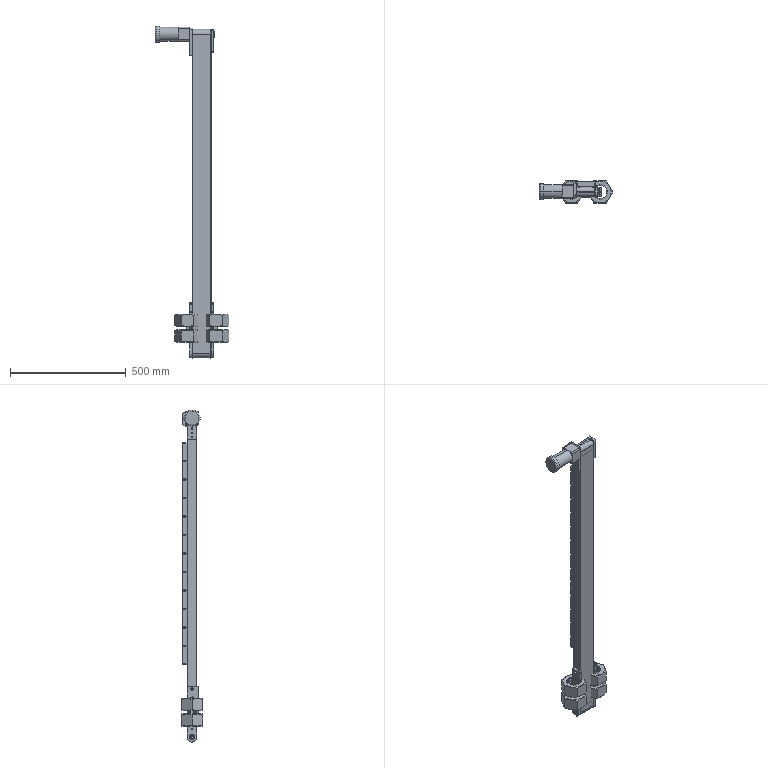Assembly | SolidWorks | mm | 36 component files | 36 solids | 1348 faces | box 318.85 x 95 x 1436.5 mm | volume 7884827 mm3 | plane 515 | cylinder 323 | cone 276 | torus 156 | sphere 78 | commonest cylinder face diameters 57.505 x112 7 x32 11 x28 5 x20 6.8 x16 6.6 x16 20.667 x12 15.333 x12
Bill of materials:
40x40X607Profile | 1 | Plain Carbon Steel | Long, slender straight bar with a uniform rectangular cross-section and no visible holes or other features.
CoilCarrier | 12 | Plain Carbon Steel | Thick, nearly square block or plate. In the face view all four corners are chamfered, and there appears to be a small rectangular notch or recess on one narrow side face.
ConveyorBelt | 1 |  | Thin, long flat strip whose narrow edges are rounded, giving a slot-like (stadium) cross-section.
ConveyorDrivenWheel | 1 | Plain Carbon Steel | Stepped, rotationally symmetric shaft or roller: a large central cylinder with a two-step smaller-diameter journal at each end, mirrored about the middle.
ConveyorDrivenWheelSidePlate | 2 | Plain Carbon Steel | Flat link plate. One end is square with chamfered corners; the other end is rounded and has a large through bore. Four smaller holes sit between them: two small holes near the chamfered corners and two medium holes on the centreline.
ConveyorDriveWheel | 1 | Plain Carbon Steel | Thick-walled hollow cylinder (sleeve or spacer-like shape) with a central axial through bore. There may be small radial holes near each end.
ConveyorDriveWheelSidePlate | 1 | Plain Carbon Steel | Flat rectangular plate with chamfered corners. Near one end it has one large through bore; three smaller holes run in a line along the centreline toward the other end.
ConveyorMotorFixingPlate | 1 | Plain Carbon Steel | Flat plate with a stepped, L-like outline: a wider end with one large through hole, then a narrower tab with three small holes in a line. A concave fillet blends the step, and the corners are chamfered.
ConveyorScrewAdjustmentSeat | 2 | Plain Carbon Steel | Rectangular block with chamfered edges. Two parallel through holes cross one large face, and a third hole enters from the top face at right angles to them, between the two.
ConveyorScrewAdjustmentSeatOne | 2 | Plain Carbon Steel | Rectangular block with chamfered edges and two parallel through holes across one large face. There is no perpendicular hole.
ConveyorSideFixedLargePlate | 1 | Plain Carbon Steel | Thick rectangular plate with chamfers on two corners along one long side. The main face has three medium holes in a line and two small holes near one end. A row of four holes is drilled into one narrow edge face.
ConveyorSideFixedLargePlateOne | 1 | Plain Carbon Steel | Thick rectangular plate almost the same as unnamed part: two chamfered corners, three centreline holes, two small end holes, and four drilled holes in one narrow edge. In the isometric view the three centreline holes look larger on the visible face.
deep groove ball bearings gb | 3 |  | Radial ball bearing shape: concentric outer and inner rings with a single row of spherical balls between them; open faces with no visible shield, seal, or cage.
hexagon nuts grade c gb | 4 |  | Hexagonal nut with a central threaded through-bore and chamfered corners on both faces.
hexagon socket head cap screws gb | 2 |  | Socket-head cap screw shape: cylindrical head with a hexagonal socket on top, above a plain cylindrical shank with a chamfered end.
Motor | 1 | Plain Carbon Steel | Compact motor-like housing: a long cylindrical body with a larger-diameter rear end cap, a square block with rounded edges at the front, and a stepped cylindrical boss with a smaller output shaft on the front face.
Mates:
1. coincident | 40x40X607Profile-1 face at (35.45, 25.646, 1510) dir (0, 1, 0) | ConveyorDrivenWheelSidePlate-3 face at (-44.55, 25.646, 235) dir (0, 1, 0)
2. distance | ConveyorDrivenWheelSidePlate-3 face at (-44.55, -14.354, 235) dir (0, 0, 1) | 40x40X607Profile-1 face at (-4.557, 5.646, 180) dir (0, 0, -1)
3. coincident | ConveyorDrivenWheelSidePlate-3 face at (-44.55, -14.354, 235) dir (0, 0, 1) | ConveyorDrivenWheelSidePlate-4 face at (35.45, 25.646, 235) dir (0, 0, 1)
4. concentric | ConveyorDrivenWheelSidePlate-3 face at (-53.55, 5.646, 155) dir (1, 0, 0) r 14 | deep groove ball bearings gb-1 face at (-42.578, 5.646, 155) dir (1, 0, 0) r 5
5. concentric | ConveyorDrivenWheelSidePlate-4 face at (44.45, 5.646, 155) dir (-1, 0, 0) r 14 | deep groove ball bearings gb-2 face at (33.479, 5.646, 155) dir (-1, 0, 0) r 5
6. coincident | ConveyorDrivenWheelSidePlate-3 face at (-53.55, 5.646, 155) dir (1, 0, 0) | deep groove ball bearings gb-1 face at (-53.55, 10.61, 142.985) dir (-1, 0, 0)
7. coincident | ConveyorDrivenWheelSidePlate-4 face at (44.45, 5.646, 155) dir (-1, 0, 0) | deep groove ball bearings gb-2 face at (44.45, 18.646, 155) dir (1, 0, 0)
8. concentric | deep groove ball bearings gb-1 face at (-42.578, 5.646, 155) dir (1, 0, 0) r 5 | ConveyorDrivenWheel-1 face at (-54.55, 5.646, 155) dir (1, 0, 0) r 7.5
9. concentric | deep groove ball bearings gb-2 face at (33.479, 5.646, 155) dir (-1, 0, 0) r 5 | ConveyorDrivenWheel-1 face at (43.45, 5.646, 155) dir (-1, 0, 0) r 7.5
10. coincident | deep groove ball bearings gb-2 face at (36.45, 13.312, 155) dir (-1, 0, 0) | ConveyorDrivenWheel-1 face at (36.45, 5.646, 155) dir (1, 0, 0)
11. concentric | ConveyorDriveWheelSidePlate-3 face at (40.45, 5.646, 1535) dir (1, 0, 0) r 14 | deep groove ball bearings gb-3 face at (51.422, 5.646, 1535) dir (1, 0, 0) r 5
12. coincident | ConveyorDriveWheelSidePlate-3 face at (40.45, 5.646, 1535) dir (1, 0, 0) | deep groove ball bearings gb-3 face at (40.45, 15.468, 1526.484) dir (-1, 0, 0)
13. concentric | deep groove ball bearings gb-3 face at (51.422, 5.646, 1535) dir (1, 0, 0) r 5 | ConveyorDriveWheel-1 face at (34.45, 5.646, 1535) dir (-1, 0, 0) r 6
14. distance | ConveyorDriveWheel-1 face at (34.45, 5.646, 1535) dir (1, 0, 0) | ConveyorDriveWheelSidePlate-3 face at (35.45, 5.646, 1505) dir (-1, 0, 0)
15. distance | ConveyorDriveWheelSidePlate-3 face at (47.45, 25.646, 1455) dir (0, 0, -1) | 40x40X607Profile-1 face at (-4.557, 5.646, 1510) dir (0, 0, 1)
16. coincident | 40x40X607Profile-1 face at (35.45, 25.646, 1510) dir (0, 1, 0) | ConveyorMotorFixingPlate-1 face at (-56.55, 25.646, 1441) dir (0, 1, 0)
17. concentric | ConveyorDriveWheel-1 face at (34.45, 5.646, 1535) dir (-1, 0, 0) r 6 | ConveyorMotorFixingPlate-1 face at (-44.55, 5.646, 1535) dir (-1, 0, 0) r 12.5
18. concentric | ConveyorDriveWheel-1 face at (34.45, 5.646, 1535) dir (-1, 0, 0) r 20.5 | ConveyorBelt-1 face at (33.45, 5.646, 1535) dir (-1, 0, 0) r 20.5
19. coincident | ConveyorDrivenWheel-1 face at (-44.55, 5.646, 155) dir (-1, 0, 0) | ConveyorBelt-1 face at (-44.55, 5.646, 1535) dir (-1, 0, 0)
20. coincident | ConveyorDrivenWheelSidePlate-3 face at (-44.55, 25.646, 235) dir (0, 1, 0) | ConveyorSideFixedLargePlate-1 face at (-44.55, 25.646, 255) dir (0, 1, 0)
21. distance | ConveyorSideFixedLargePlate-1 face at (-44.55, -20.354, 255) dir (0, 0, -1) | ConveyorDrivenWheelSidePlate-3 face at (-44.55, -14.354, 235) dir (0, 0, 1)
22. coincident | ConveyorDrivenWheelSidePlate-4 face at (35.45, 25.646, 235) dir (0, 1, 0) | ConveyorSideFixedLargePlateOne-2 face at (47.45, 25.646, 255) dir (0, 1, 0)
23. distance | ConveyorSideFixedLargePlateOne-2 face at (47.45, -20.354, 255) dir (0, 0, -1) | ConveyorDrivenWheelSidePlate-4 face at (35.45, 25.646, 235) dir (0, 0, 1)
24. concentric | ConveyorDrivenWheelSidePlate-3 face at (-56.55, 17.646, 227.5) dir (-1, 0, 0) r 2.5 | ConveyorScrewAdjustmentSeatOne-1 face at (-72.55, 17.646, 227.5) dir (-1, 0, 0) r 5.5
25. concentric | ConveyorDrivenWheelSidePlate-3 face at (-56.55, -6.354, 227.5) dir (-1, 0, 0) r 2.5 | ConveyorScrewAdjustmentSeatOne-1 face at (-72.55, -6.354, 227.5) dir (-1, 0, 0) r 5.5
26. coincident | ConveyorDrivenWheelSidePlate-3 face at (-56.55, 5.646, 185) dir (-1, 0, 0) | ConveyorScrewAdjustmentSeatOne-1 face at (-56.55, 5.646, 227.5) dir (1, 0, 0)
27. concentric | ConveyorSideFixedLargePlate-1 face at (-56.55, 17.646, 262.5) dir (-1, 0, 0) r 2.5 | ConveyorScrewAdjustmentSeat-1 face at (-72.55, 17.646, 262.5) dir (-1, 0, 0) r 5.5
28. concentric | ConveyorSideFixedLargePlate-1 face at (-56.55, -6.354, 262.5) dir (-1, 0, 0) r 2.5 | ConveyorScrewAdjustmentSeat-1 face at (-72.55, -6.354, 262.5) dir (-1, 0, 0) r 5.5
29. coincident | ConveyorSideFixedLargePlate-1 face at (-56.55, 2.646, 315) dir (-1, 0, 0) | ConveyorScrewAdjustmentSeat-1 face at (-56.55, 5.646, 262.5) dir (1, 0, 0)
30. concentric | ConveyorSideFixedLargePlateOne-2 face at (35.45, 17.646, 262.5) dir (-1, 0, 0) r 2.5 | ConveyorScrewAdjustmentSeat-2 face at (63.45, 17.646, 262.5) dir (1, 0, 0) r 5.5
31. concentric | ConveyorSideFixedLargePlateOne-2 face at (35.45, -6.354, 262.5) dir (-1, 0, 0) r 2.5 | ConveyorScrewAdjustmentSeat-2 face at (63.45, -6.354, 262.5) dir (1, 0, 0) r 5.5
32. coincident | ConveyorSideFixedLargePlateOne-2 face at (47.45, 2.646, 315) dir (1, 0, 0) | ConveyorScrewAdjustmentSeat-2 face at (47.45, 5.646, 262.5) dir (-1, 0, 0)
33. concentric | ConveyorDrivenWheelSidePlate-4 face at (47.45, 17.646, 227.5) dir (1, 0, 0) r 2.5 | ConveyorScrewAdjustmentSeatOne-2 face at (63.45, 17.646, 227.5) dir (1, 0, 0) r 5.5
34. concentric | ConveyorDrivenWheelSidePlate-4 face at (47.45, -6.354, 227.5) dir (1, 0, 0) r 2.5 | ConveyorScrewAdjustmentSeatOne-2 face at (63.45, -6.354, 227.5) dir (1, 0, 0) r 5.5
35. coincident | ConveyorDrivenWheelSidePlate-4 face at (47.45, 5.646, 185) dir (1, 0, 0) | ConveyorScrewAdjustmentSeatOne-2 face at (47.45, 5.646, 227.5) dir (-1, 0, 0)
36. concentric | ConveyorScrewAdjustmentSeat-2 face at (57.45, 5.646, 270) dir (0, 0, 1) r 4 | hexagon socket head cap screws gb-1 face at (57.45, 5.646, 279) dir (0, 0, 1) r 0.8
37. distance | ConveyorScrewAdjustmentSeat-2 face at (63.45, -14.354, 270) dir (0, 0, 1) | hexagon socket head cap screws gb-1 face at (57.45, 5.646, 285) dir (0, 0, -1)
38. concentric | ConveyorScrewAdjustmentSeat-1 face at (-66.55, 5.646, 270) dir (0, 0, 1) r 4 | hexagon socket head cap screws gb-2 face at (-66.55, 5.646, 279) dir (0, 0, 1) r 0.8
39. distance | ConveyorScrewAdjustmentSeat-1 face at (-72.55, 25.646, 270) dir (0, 0, 1) | hexagon socket head cap screws gb-2 face at (-66.55, 5.646, 285) dir (0, 0, -1)
40. concentric | hexagon socket head cap screws gb-1 face at (57.45, 5.646, 279) dir (0, 0, 1) r 0.8 | hexagon nuts grade c gb-1 face at (57.45, 5.646, 270) dir (0, 0, 1) r 28.753
41. concentric | hexagon socket head cap screws gb-1 face at (57.45, 5.646, 279) dir (0, 0, 1) r 0.8 | hexagon nuts grade c gb-2 face at (57.45, 5.646, 202.6) dir (0, 0, 1) r 28.753
42. concentric | hexagon socket head cap screws gb-2 face at (-66.55, 5.646, 279) dir (0, 0, 1) r 0.8 | hexagon nuts grade c gb-3 face at (-66.55, 5.646, 202.6) dir (0, 0, 1) r 28.753
43. concentric | hexagon socket head cap screws gb-2 face at (-66.55, 5.646, 279) dir (0, 0, 1) r 0.8 | hexagon nuts grade c gb-4 face at (-66.55, 5.646, 270) dir (0, 0, 1) r 28.753
44. coincident | ConveyorScrewAdjustmentSeat-1 face at (-72.55, 25.646, 270) dir (0, 0, 1) | hexagon nuts grade c gb-4 face at (-39.125, -41.854, 270) dir (0, 0, -1)
45. coincident | ConveyorScrewAdjustmentSeat-1 face at (-72.55, 25.646, 255) dir (0, 0, -1) | hexagon nuts grade c gb-3 face at (-39.125, -41.854, 255) dir (0, 0, 1)
46. coincident | ConveyorScrewAdjustmentSeat-2 face at (63.45, -14.354, 270) dir (0, 0, 1) | hexagon nuts grade c gb-1 face at (84.875, -41.854, 270) dir (0, 0, -1)
47. coincident | ConveyorScrewAdjustmentSeat-2 face at (63.45, -14.354, 255) dir (0, 0, -1) | hexagon nuts grade c gb-2 face at (84.875, -41.854, 255) dir (0, 0, 1)
48. coincident | 40x40X607Profile-1 face at (35.45, -14.354, 1510) dir (1, 0, 0) | ConveyorDriveWheelSidePlate-3 face at (35.45, 5.646, 1505) dir (-1, 0, 0)
49. coincident | 40x40X607Profile-1 face at (-44.55, -14.354, 1510) dir (-1, 0, 0) | ConveyorMotorFixingPlate-1 face at (-44.55, 5.646, 1501) dir (1, 0, 0)
50. coincident | 40x40X607Profile-1 face at (-44.55, -14.354, 1510) dir (-1, 0, 0) | ConveyorDrivenWheelSidePlate-3 face at (-44.55, 5.646, 185) dir (1, 0, 0)
51. coincident | 40x40X607Profile-1 face at (35.45, -14.354, 1510) dir (1, 0, 0) | ConveyorDrivenWheelSidePlate-4 face at (35.45, 5.646, 185) dir (-1, 0, 0)
52. coincident | 40x40X607Profile-1 face at (-44.55, -14.354, 1510) dir (-1, 0, 0) | ConveyorSideFixedLargePlate-1 face at (-44.55, 2.646, 315) dir (1, 0, 0)
53. coincident | 40x40X607Profile-1 face at (35.45, -14.354, 1510) dir (1, 0, 0) | ConveyorSideFixedLargePlateOne-2 face at (35.45, 2.646, 315) dir (-1, 0, 0)
54. concentric | ConveyorMotorFixingPlate-1 face at (-44.55, 5.646, 1535) dir (-1, 0, 0) r 12.5 | Motor-1 face at (-23.55, 5.646, 1535) dir (-1, 0, 0) r 6
55. coincident | ConveyorMotorFixingPlate-1 face at (-56.55, 5.646, 1501) dir (-1, 0, 0) | Motor-1 face at (-56.55, 5.646, 1535) dir (1, 0, 0)
56. parallel | ConveyorMotorFixingPlate-1 face at (-56.55, 45.646, 1501) dir (0, 1, 0) | Motor-1 face at (-56.55, 35.646, 1505) dir (0, 1, 0)
57. coincident | ConveyorBelt-1 face at (33.45, 27.146, 1535) dir (0, 1, 0) | CoilCarrier-1 face at (-4.55, 27.146, 1388.775) dir (0, -1, 0)
58. coincident | 40x40X607Profile-1 face at (35.45, -14.354, 1510) dir (1, 0, 0) | CoilCarrier-1 face at (35.45, 47.146, 1348.775) dir (1, 0, 0)
59. parallel | 40x40X607Profile-1 face at (35.45, 25.646, 1510) dir (0, 1, 0) | ConveyorBelt-1 face at (33.45, 27.146, 1535) dir (0, 1, 0)